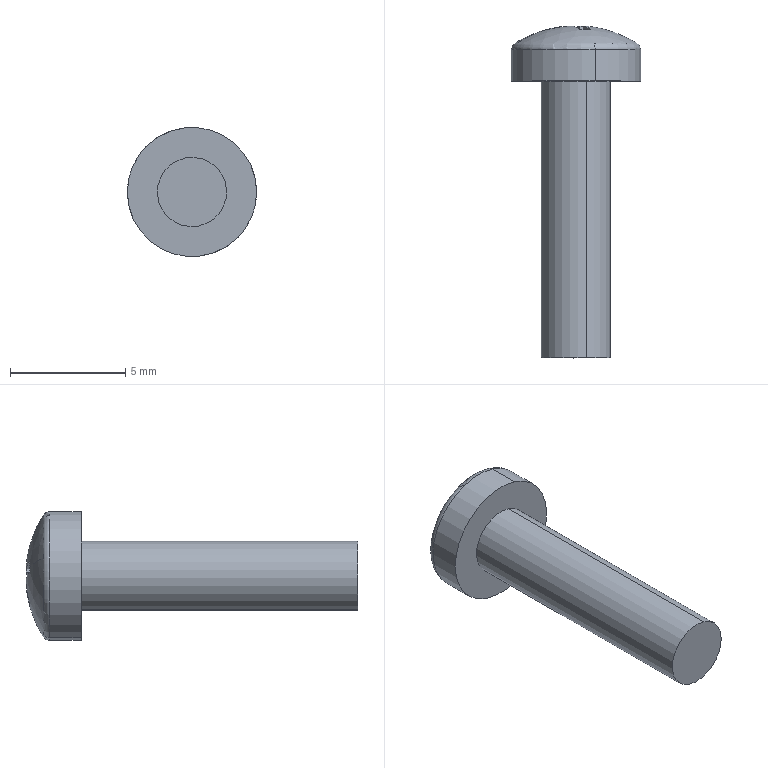Component | SolidWorks | pan cross head_am_pkg-1 | 1 solid | 23 faces | box 5.6 x 14.39 x 5.6 mm | volume 132 mm3 | plane 15 | cylinder 4 | torus 2 | sphere 2 | commonest cylinder face diameters 5.6 x2 3 x2
STEP:
#1=COLOUR_RGB('',0.7922,0.8196,0.9333);
#2=FILL_AREA_STYLE_COLOUR('',#1);
#3=FILL_AREA_STYLE('',(#2));
#4=SURFACE_STYLE_FILL_AREA(#3);
#5=SURFACE_SIDE_STYLE('',(#4));
#6=SURFACE_STYLE_USAGE(.BOTH.,#5);
#7=PRESENTATION_STYLE_ASSIGNMENT((#6));
#8=CARTESIAN_POINT('',(0.5678,0.5654,-0.7057));
#9=VERTEX_POINT('',#8);
#10=CARTESIAN_POINT('',(0.633,0.5654,-0.4951));
#11=VERTEX_POINT('',#10);
#12=CARTESIAN_POINT('',(0.6004,0.5654,-0.6004));
#13=DIRECTION('',(0.,1.,-0.));
#14=DIRECTION('',(-0.2959,0.,-0.9552));
#15=AXIS2_PLACEMENT_3D('',#12,#13,#14);
#16=CIRCLE('',#15,0.1102);
#17=EDGE_CURVE('',#9,#11,#16,.T.);
#18=ORIENTED_EDGE('',*,*,#17,.T.);
#19=CARTESIAN_POINT('',(0.6312,0.5766,-0.5011));
#20=VERTEX_POINT('',#19);
#21=CARTESIAN_POINT('',(0.6291,0.5654,-0.5077));
#22=DIRECTION('',(-0.9552,0.,0.2959));
#23=DIRECTION('',(0.2959,0.,0.9552));
#24=AXIS2_PLACEMENT_3D('',#21,#22,#23);
#25=CIRCLE('',#24,0.01323);
#26=EDGE_CURVE('',#11,#20,#25,.T.);
#27=ORIENTED_EDGE('',*,*,#26,.T.);
#28=CARTESIAN_POINT('',(0.5011,0.5766,-0.5696));
#29=VERTEX_POINT('',#28);
#30=CARTESIAN_POINT('',(0.6004,0.5766,-0.6004));
#31=DIRECTION('',(0.,1.,-0.));
#32=DIRECTION('',(-0.2959,0.,-0.9552));
#33=AXIS2_PLACEMENT_3D('',#30,#31,#32);
#34=CIRCLE('',#33,0.104);
#35=EDGE_CURVE('',#29,#20,#34,.T.);
#36=ORIENTED_EDGE('',*,*,#35,.F.);
#37=CARTESIAN_POINT('',(0.5696,0.5766,-0.6997));
#38=VERTEX_POINT('',#37);
#39=CARTESIAN_POINT('',(0.6004,0.5766,-0.6004));
#40=DIRECTION('',(0.,1.,-0.));
#41=DIRECTION('',(-0.2959,0.,-0.9552));
#42=AXIS2_PLACEMENT_3D('',#39,#40,#41);
#43=CIRCLE('',#42,0.104);
#44=EDGE_CURVE('',#38,#29,#43,.T.);
#45=ORIENTED_EDGE('',*,*,#44,.F.);
#46=CARTESIAN_POINT('',(0.5717,0.5654,-0.6931));
#47=DIRECTION('',(0.9552,-0.,-0.2959));
#48=DIRECTION('',(-0.2959,0.,-0.9552));
#49=AXIS2_PLACEMENT_3D('',#46,#47,#48);
#50=CIRCLE('',#49,0.01323);
#51=EDGE_CURVE('',#9,#38,#50,.T.);
#52=ORIENTED_EDGE('',*,*,#51,.F.);
#53=EDGE_LOOP('',(#18,#27,#36,#45,#52));
#54=FACE_OUTER_BOUND('',#53,.T.);
#55=CARTESIAN_POINT('',(0.6004,0.5654,-0.6004));
#56=DIRECTION('',(0.,1.,-0.));
#57=DIRECTION('',(-0.2959,-0.,-0.9552));
#58=AXIS2_PLACEMENT_3D('',#55,#56,#57);
#59=TOROIDAL_SURFACE('',#58,0.09701,0.01323);
#60=ADVANCED_FACE('',(#54),#59,.T.);
#61=CARTESIAN_POINT('',(0.5678,0.5118,-0.7057));
#62=VERTEX_POINT('',#61);
#63=CARTESIAN_POINT('',(0.633,0.5118,-0.4951));
#64=VERTEX_POINT('',#63);
#65=CARTESIAN_POINT('',(0.6004,0.5118,-0.6004));
#66=DIRECTION('',(0.,1.,-0.));
#67=DIRECTION('',(-0.2959,0.,-0.9552));
#68=AXIS2_PLACEMENT_3D('',#65,#66,#67);
#69=CIRCLE('',#68,0.1102);
#70=EDGE_CURVE('',#62,#64,#69,.T.);
#71=ORIENTED_EDGE('',*,*,#70,.T.);
#72=CARTESIAN_POINT('',(0.633,1.606,-0.4951));
#73=DIRECTION('',(0.,1.,-0.));
#74=VECTOR('',#73,39.37);
#75=LINE('',#72,#74);
#76=EDGE_CURVE('',#64,#11,#75,.T.);
#77=ORIENTED_EDGE('',*,*,#76,.T.);
#78=ORIENTED_EDGE('',*,*,#17,.F.);
#79=CARTESIAN_POINT('',(0.5678,1.606,-0.7057));
#80=DIRECTION('',(0.,1.,-0.));
#81=VECTOR('',#80,39.37);
#82=LINE('',#79,#81);
#83=EDGE_CURVE('',#62,#9,#82,.T.);
#84=ORIENTED_EDGE('',*,*,#83,.F.);
#85=EDGE_LOOP('',(#71,#77,#78,#84));
#86=FACE_OUTER_BOUND('',#85,.T.);
#87=CARTESIAN_POINT('',(0.6004,1.606,-0.6004));
#88=DIRECTION('',(0.,1.,-0.));
#89=DIRECTION('',(-0.2959,0.,-0.9552));
#90=AXIS2_PLACEMENT_3D('',#87,#88,#89);
#91=CYLINDRICAL_SURFACE('',#90,0.1102);
#92=ADVANCED_FACE('',(#86),#91,.T.);
#93=CARTESIAN_POINT('',(0.5829,0.03937,-0.6568));
#94=VERTEX_POINT('',#93);
#95=CARTESIAN_POINT('',(0.6179,0.03937,-0.544));
#96=VERTEX_POINT('',#95);
#97=CARTESIAN_POINT('',(0.6004,0.03937,-0.6004));
#98=DIRECTION('',(0.,1.,-0.));
#99=DIRECTION('',(-0.2959,-0.,-0.9552));
#100=AXIS2_PLACEMENT_3D('',#97,#98,#99);
#101=CIRCLE('',#100,0.05906);
#102=EDGE_CURVE('',#94,#96,#101,.T.);
#103=ORIENTED_EDGE('',*,*,#102,.T.);
#104=CARTESIAN_POINT('',(0.6179,0.5118,-0.544));
#105=VERTEX_POINT('',#104);
#106=CARTESIAN_POINT('',(0.6179,1.606,-0.544));
#107=DIRECTION('',(0.,1.,-0.));
#108=VECTOR('',#107,39.37);
#109=LINE('',#106,#108);
#110=EDGE_CURVE('',#96,#105,#109,.T.);
#111=ORIENTED_EDGE('',*,*,#110,.T.);
#112=CARTESIAN_POINT('',(0.5829,0.5118,-0.6568));
#113=VERTEX_POINT('',#112);
#114=CARTESIAN_POINT('',(0.6004,0.5118,-0.6004));
#115=DIRECTION('',(0.,1.,-0.));
#116=DIRECTION('',(-0.2959,0.,-0.9552));
#117=AXIS2_PLACEMENT_3D('',#114,#115,#116);
#118=CIRCLE('',#117,0.05906);
#119=EDGE_CURVE('',#113,#105,#118,.T.);
#120=ORIENTED_EDGE('',*,*,#119,.F.);
#121=CARTESIAN_POINT('',(0.5829,1.606,-0.6568));
#122=DIRECTION('',(0.,1.,-0.));
#123=VECTOR('',#122,39.37);
#124=LINE('',#121,#123);
#125=EDGE_CURVE('',#94,#113,#124,.T.);
#126=ORIENTED_EDGE('',*,*,#125,.F.);
#127=EDGE_LOOP('',(#103,#111,#120,#126));
#128=FACE_OUTER_BOUND('',#127,.T.);
#129=CARTESIAN_POINT('',(0.6004,1.606,-0.6004));
#130=DIRECTION('',(0.,1.,-0.));
#131=DIRECTION('',(-0.2959,0.,-0.9552));
#132=AXIS2_PLACEMENT_3D('',#129,#130,#131);
#133=CYLINDRICAL_SURFACE('',#132,0.05906);
#134=ADVANCED_FACE('',(#128),#133,.T.);
#135=ORIENTED_EDGE('',*,*,#35,.T.);
#136=CARTESIAN_POINT('',(0.6997,0.5766,-0.6312));
#137=VERTEX_POINT('',#136);
#138=CARTESIAN_POINT('',(0.6004,0.5766,-0.6004));
#139=DIRECTION('',(0.,1.,-0.));
#140=DIRECTION('',(-0.2959,0.,-0.9552));
#141=AXIS2_PLACEMENT_3D('',#138,#139,#140);
#142=CIRCLE('',#141,0.104);
#143=EDGE_CURVE('',#20,#137,#142,.T.);
#144=ORIENTED_EDGE('',*,*,#143,.T.);
#145=CARTESIAN_POINT('',(0.6496,0.5994,-0.6156));
#146=VERTEX_POINT('',#145);
#147=CARTESIAN_POINT('',(0.6004,0.4094,-0.6004));
#148=DIRECTION('',(0.2959,0.,0.9552));
#149=DIRECTION('',(0.9552,0.,-0.2959));
#150=AXIS2_PLACEMENT_3D('',#147,#148,#149);
#151=CIRCLE('',#150,0.1969);
#152=EDGE_CURVE('',#137,#146,#151,.T.);
#153=ORIENTED_EDGE('',*,*,#152,.T.);
#154=CARTESIAN_POINT('',(0.6524,0.5992,-0.6064));
#155=VERTEX_POINT('',#154);
#156=CARTESIAN_POINT('',(0.5508,0.4439,-0.585));
#157=DIRECTION('',(0.7954,-0.5538,-0.2464));
#158=DIRECTION('',(-0.529,-0.8327,0.1639));
#159=AXIS2_PLACEMENT_3D('',#156,#157,#158);
#160=CIRCLE('',#159,0.1867);
#161=EDGE_CURVE('',#146,#155,#160,.T.);
#162=ORIENTED_EDGE('',*,*,#161,.T.);
#163=CARTESIAN_POINT('',(0.613,0.6058,-0.5937));
#164=VERTEX_POINT('',#163);
#165=CARTESIAN_POINT('',(0.5995,0.4096,-0.6031));
#166=DIRECTION('',(-0.2952,0.06592,-0.9531));
#167=DIRECTION('',(-0.0195,-0.9978,-0.06296));
#168=AXIS2_PLACEMENT_3D('',#165,#166,#167);
#169=CIRCLE('',#168,0.1968);
#170=EDGE_CURVE('',#164,#155,#169,.T.);
#171=ORIENTED_EDGE('',*,*,#170,.F.);
#172=CARTESIAN_POINT('',(0.6248,0.5992,-0.5542));
#173=VERTEX_POINT('',#172);
#174=CARTESIAN_POINT('',(0.5977,0.4096,-0.5995));
#175=DIRECTION('',(-0.9531,0.06592,0.2952));
#176=DIRECTION('',(0.06296,0.9978,-0.0195));
#177=AXIS2_PLACEMENT_3D('',#174,#175,#176);
#178=CIRCLE('',#177,0.1968);
#179=EDGE_CURVE('',#173,#164,#178,.T.);
#180=ORIENTED_EDGE('',*,*,#179,.F.);
#181=CARTESIAN_POINT('',(0.6064,0.5992,-0.5484));
#182=VERTEX_POINT('',#181);
#183=CARTESIAN_POINT('',(0.585,0.4439,-0.6499));
#184=DIRECTION('',(0.2464,-0.5538,0.7954));
#185=DIRECTION('',(0.1639,0.8327,0.529));
#186=AXIS2_PLACEMENT_3D('',#183,#184,#185);
#187=CIRCLE('',#186,0.1867);
#188=EDGE_CURVE('',#173,#182,#187,.T.);
#189=ORIENTED_EDGE('',*,*,#188,.T.);
#190=CARTESIAN_POINT('',(0.5937,0.6058,-0.5878));
#191=VERTEX_POINT('',#190);
#192=CARTESIAN_POINT('',(0.6031,0.4096,-0.6012));
#193=DIRECTION('',(0.9531,0.06592,-0.2952));
#194=DIRECTION('',(0.06296,-0.9978,-0.0195));
#195=AXIS2_PLACEMENT_3D('',#192,#193,#194);
#196=CIRCLE('',#195,0.1968);
#197=EDGE_CURVE('',#191,#182,#196,.T.);
#198=ORIENTED_EDGE('',*,*,#197,.F.);
#199=CARTESIAN_POINT('',(0.5542,0.5992,-0.5759));
#200=VERTEX_POINT('',#199);
#201=CARTESIAN_POINT('',(0.5995,0.4096,-0.6031));
#202=DIRECTION('',(-0.2952,0.06592,-0.9531));
#203=DIRECTION('',(-0.0195,-0.9978,-0.06296));
#204=AXIS2_PLACEMENT_3D('',#201,#202,#203);
#205=CIRCLE('',#204,0.1968);
#206=EDGE_CURVE('',#200,#191,#205,.T.);
#207=ORIENTED_EDGE('',*,*,#206,.F.);
#208=CARTESIAN_POINT('',(0.5512,0.5994,-0.5851));
#209=VERTEX_POINT('',#208);
#210=CARTESIAN_POINT('',(0.6499,0.4439,-0.6157));
#211=DIRECTION('',(-0.7954,-0.5538,0.2464));
#212=DIRECTION('',(-0.529,0.8327,0.1639));
#213=AXIS2_PLACEMENT_3D('',#210,#211,#212);
#214=CIRCLE('',#213,0.1867);
#215=EDGE_CURVE('',#200,#209,#214,.T.);
#216=ORIENTED_EDGE('',*,*,#215,.T.);
#217=CARTESIAN_POINT('',(0.6004,0.4094,-0.6004));
#218=DIRECTION('',(-0.2959,-0.,-0.9552));
#219=DIRECTION('',(-0.9552,0.,0.2959));
#220=AXIS2_PLACEMENT_3D('',#217,#218,#219);
#221=CIRCLE('',#220,0.1969);
#222=EDGE_CURVE('',#29,#209,#221,.T.);
#223=ORIENTED_EDGE('',*,*,#222,.F.);
#224=EDGE_LOOP('',(#135,#144,#153,#162,#171,#180,#189,#198,#207,#216,#223));
#225=FACE_OUTER_BOUND('',#224,.T.);
#226=CARTESIAN_POINT('',(0.6004,0.4094,-0.6004));
#227=DIRECTION('',(0.2959,0.,0.9552));
#228=DIRECTION('',(-0.9552,0.,0.2959));
#229=AXIS2_PLACEMENT_3D('',#226,#227,#228);
#230=SPHERICAL_SURFACE('',#229,0.1969);
#231=ADVANCED_FACE('',(#225),#230,.T.);
#232=ORIENTED_EDGE('',*,*,#152,.F.);
#233=CARTESIAN_POINT('',(0.6004,0.5766,-0.6004));
#234=DIRECTION('',(0.,1.,-0.));
#235=DIRECTION('',(-0.2959,0.,-0.9552));
#236=AXIS2_PLACEMENT_3D('',#233,#234,#235);
#237=CIRCLE('',#236,0.104);
#238=EDGE_CURVE('',#137,#38,#237,.T.);
#239=ORIENTED_EDGE('',*,*,#238,.T.);
#240=ORIENTED_EDGE('',*,*,#44,.T.);
#241=ORIENTED_EDGE('',*,*,#222,.T.);
#242=CARTESIAN_POINT('',(0.5484,0.5992,-0.5944));
#243=VERTEX_POINT('',#242);
#244=CARTESIAN_POINT('',(0.6499,0.4439,-0.6157));
#245=DIRECTION('',(-0.7954,-0.5538,0.2464));
#246=DIRECTION('',(-0.529,0.8327,0.1639));
#247=AXIS2_PLACEMENT_3D('',#244,#245,#246);
#248=CIRCLE('',#247,0.1867);
#249=EDGE_CURVE('',#209,#243,#248,.T.);
#250=ORIENTED_EDGE('',*,*,#249,.T.);
#251=CARTESIAN_POINT('',(0.5878,0.6058,-0.6071));
#252=VERTEX_POINT('',#251);
#253=CARTESIAN_POINT('',(0.6012,0.4096,-0.5977));
#254=DIRECTION('',(0.2952,0.06592,0.9531));
#255=DIRECTION('',(-0.0195,0.9978,-0.06296));
#256=AXIS2_PLACEMENT_3D('',#253,#254,#255);
#257=CIRCLE('',#256,0.1968);
#258=EDGE_CURVE('',#252,#243,#257,.T.);
#259=ORIENTED_EDGE('',*,*,#258,.F.);
#260=CARTESIAN_POINT('',(0.5759,0.5992,-0.6466));
#261=VERTEX_POINT('',#260);
#262=CARTESIAN_POINT('',(0.6031,0.4096,-0.6012));
#263=DIRECTION('',(0.9531,0.06592,-0.2952));
#264=DIRECTION('',(0.06296,-0.9978,-0.0195));
#265=AXIS2_PLACEMENT_3D('',#262,#263,#264);
#266=CIRCLE('',#265,0.1968);
#267=EDGE_CURVE('',#261,#252,#266,.T.);
#268=ORIENTED_EDGE('',*,*,#267,.F.);
#269=CARTESIAN_POINT('',(0.5944,0.5992,-0.6524));
#270=VERTEX_POINT('',#269);
#271=CARTESIAN_POINT('',(0.6157,0.4439,-0.5508));
#272=DIRECTION('',(-0.2464,-0.5538,-0.7954));
#273=DIRECTION('',(0.1639,-0.8327,0.529));
#274=AXIS2_PLACEMENT_3D('',#271,#272,#273);
#275=CIRCLE('',#274,0.1867);
#276=EDGE_CURVE('',#261,#270,#275,.T.);
#277=ORIENTED_EDGE('',*,*,#276,.T.);
#278=CARTESIAN_POINT('',(0.6071,0.6058,-0.613));
#279=VERTEX_POINT('',#278);
#280=CARTESIAN_POINT('',(0.5977,0.4096,-0.5995));
#281=DIRECTION('',(-0.9531,0.06592,0.2952));
#282=DIRECTION('',(0.06296,0.9978,-0.0195));
#283=AXIS2_PLACEMENT_3D('',#280,#281,#282);
#284=CIRCLE('',#283,0.1968);
#285=EDGE_CURVE('',#279,#270,#284,.T.);
#286=ORIENTED_EDGE('',*,*,#285,.F.);
#287=CARTESIAN_POINT('',(0.6466,0.5992,-0.6248));
#288=VERTEX_POINT('',#287);
#289=CARTESIAN_POINT('',(0.6012,0.4096,-0.5977));
#290=DIRECTION('',(0.2952,0.06592,0.9531));
#291=DIRECTION('',(-0.0195,0.9978,-0.06296));
#292=AXIS2_PLACEMENT_3D('',#289,#290,#291);
#293=CIRCLE('',#292,0.1968);
#294=EDGE_CURVE('',#288,#279,#293,.T.);
#295=ORIENTED_EDGE('',*,*,#294,.F.);
#296=CARTESIAN_POINT('',(0.5508,0.4439,-0.585));
#297=DIRECTION('',(0.7954,-0.5538,-0.2464));
#298=DIRECTION('',(-0.529,-0.8327,0.1639));
#299=AXIS2_PLACEMENT_3D('',#296,#297,#298);
#300=CIRCLE('',#299,0.1867);
#301=EDGE_CURVE('',#288,#146,#300,.T.);
#302=ORIENTED_EDGE('',*,*,#301,.T.);
#303=EDGE_LOOP('',(#232,#239,#240,#241,#250,#259,#268,#277,#286,#295,#302));
#304=FACE_OUTER_BOUND('',#303,.T.);
#305=CARTESIAN_POINT('',(0.6004,0.4094,-0.6004));
#306=DIRECTION('',(0.2959,0.,0.9552));
#307=DIRECTION('',(-0.9552,0.,0.2959));
#308=AXIS2_PLACEMENT_3D('',#305,#306,#307);
#309=SPHERICAL_SURFACE('',#308,0.1969);
#310=ADVANCED_FACE('',(#304),#309,.T.);
#311=ORIENTED_EDGE('',*,*,#206,.T.);
#312=CARTESIAN_POINT('',(0.5971,0.5296,-0.5941));
#313=VERTEX_POINT('',#312);
#314=CARTESIAN_POINT('',(0.5974,0.5216,-0.5947));
#315=DIRECTION('',(0.04337,-0.9957,-0.08229));
#316=VECTOR('',#315,39.37);
#317=LINE('',#314,#316);
#318=EDGE_CURVE('',#191,#313,#317,.T.);
#319=ORIENTED_EDGE('',*,*,#318,.T.);
#320=CARTESIAN_POINT('',(0.5498,0.6063,-0.5741));
#321=DIRECTION('',(0.5119,-0.8314,-0.2161));
#322=VECTOR('',#321,39.37);
#323=LINE('',#320,#322);
#324=EDGE_CURVE('',#200,#313,#323,.T.);
#325=ORIENTED_EDGE('',*,*,#324,.F.);
#326=EDGE_LOOP('',(#311,#319,#325));
#327=FACE_OUTER_BOUND('',#326,.T.);
#328=CARTESIAN_POINT('',(0.6017,0.5219,-0.596));
#329=DIRECTION('',(-0.2952,0.06592,-0.9531));
#330=DIRECTION('',(-0.0195,-0.9978,-0.06296));
#331=AXIS2_PLACEMENT_3D('',#328,#329,#330);
#332=PLANE('',#331);
#333=ADVANCED_FACE('',(#327),#332,.T.);
#334=CARTESIAN_POINT('',(0.6067,0.5296,-0.5971));
#335=VERTEX_POINT('',#334);
#336=CARTESIAN_POINT('',(0.657,0.6063,-0.6073));
#337=DIRECTION('',(-0.5444,-0.8314,0.1111));
#338=VECTOR('',#337,39.37);
#339=LINE('',#336,#338);
#340=EDGE_CURVE('',#155,#335,#339,.T.);
#341=ORIENTED_EDGE('',*,*,#340,.T.);
#342=CARTESIAN_POINT('',(0.6061,0.5216,-0.5974));
#343=DIRECTION('',(0.08229,0.9957,0.04337));
#344=VECTOR('',#343,39.37);
#345=LINE('',#342,#344);
#346=EDGE_CURVE('',#335,#164,#345,.T.);
#347=ORIENTED_EDGE('',*,*,#346,.T.);
#348=ORIENTED_EDGE('',*,*,#170,.T.);
#349=EDGE_LOOP('',(#341,#347,#348));
#350=FACE_OUTER_BOUND('',#349,.T.);
#351=CARTESIAN_POINT('',(0.6017,0.5219,-0.596));
#352=DIRECTION('',(-0.2952,0.06592,-0.9531));
#353=DIRECTION('',(-0.0195,-0.9978,-0.06296));
#354=AXIS2_PLACEMENT_3D('',#351,#352,#353);
#355=PLANE('',#354);
#356=ADVANCED_FACE('',(#350),#355,.T.);
#357=CARTESIAN_POINT('',(0.5941,0.5296,-0.6037));
#358=VERTEX_POINT('',#357);
#359=CARTESIAN_POINT('',(0.5438,0.6063,-0.5935));
#360=DIRECTION('',(0.5444,-0.8314,-0.1111));
#361=VECTOR('',#360,39.37);
#362=LINE('',#359,#361);
#363=EDGE_CURVE('',#243,#358,#362,.T.);
#364=ORIENTED_EDGE('',*,*,#363,.T.);
#365=CARTESIAN_POINT('',(0.5947,0.5216,-0.6034));
#366=DIRECTION('',(-0.08229,0.9957,-0.04337));
#367=VECTOR('',#366,39.37);
#368=LINE('',#365,#367);
#369=EDGE_CURVE('',#358,#252,#368,.T.);
#370=ORIENTED_EDGE('',*,*,#369,.T.);
#371=ORIENTED_EDGE('',*,*,#258,.T.);
#372=EDGE_LOOP('',(#364,#370,#371));
#373=FACE_OUTER_BOUND('',#372,.T.);
#374=CARTESIAN_POINT('',(0.599,0.5219,-0.6048));
#375=DIRECTION('',(0.2952,0.06592,0.9531));
#376=DIRECTION('',(-0.0195,0.9978,-0.06296));
#377=AXIS2_PLACEMENT_3D('',#374,#375,#376);
#378=PLANE('',#377);
#379=ADVANCED_FACE('',(#373),#378,.T.);
#380=ORIENTED_EDGE('',*,*,#294,.T.);
#381=CARTESIAN_POINT('',(0.6037,0.5296,-0.6067));
#382=VERTEX_POINT('',#381);
#383=CARTESIAN_POINT('',(0.6034,0.5216,-0.6061));
#384=DIRECTION('',(-0.04337,-0.9957,0.08229));
#385=VECTOR('',#384,39.37);
#386=LINE('',#383,#385);
#387=EDGE_CURVE('',#279,#382,#386,.T.);
#388=ORIENTED_EDGE('',*,*,#387,.T.);
#389=CARTESIAN_POINT('',(0.651,0.6063,-0.6267));
#390=DIRECTION('',(-0.5119,-0.8314,0.2161));
#391=VECTOR('',#390,39.37);
#392=LINE('',#389,#391);
#393=EDGE_CURVE('',#288,#382,#392,.T.);
#394=ORIENTED_EDGE('',*,*,#393,.F.);
#395=EDGE_LOOP('',(#380,#388,#394));
#396=FACE_OUTER_BOUND('',#395,.T.);
#397=CARTESIAN_POINT('',(0.599,0.5219,-0.6048));
#398=DIRECTION('',(0.2952,0.06592,0.9531));
#399=DIRECTION('',(-0.0195,0.9978,-0.06296));
#400=AXIS2_PLACEMENT_3D('',#397,#398,#399);
#401=PLANE('',#400);
#402=ADVANCED_FACE('',(#396),#401,.T.);
#403=ORIENTED_EDGE('',*,*,#110,.F.);
#404=CARTESIAN_POINT('',(0.6004,0.03937,-0.6004));
#405=DIRECTION('',(0.,1.,-0.));
#406=DIRECTION('',(-0.2959,-0.,-0.9552));
#407=AXIS2_PLACEMENT_3D('',#404,#405,#406);
#408=CIRCLE('',#407,0.05906);
#409=EDGE_CURVE('',#96,#94,#408,.T.);
#410=ORIENTED_EDGE('',*,*,#409,.T.);
#411=ORIENTED_EDGE('',*,*,#125,.T.);
#412=CARTESIAN_POINT('',(0.6004,0.5118,-0.6004));
#413=DIRECTION('',(0.,1.,-0.));
#414=DIRECTION('',(-0.2959,0.,-0.9552));
#415=AXIS2_PLACEMENT_3D('',#412,#413,#414);
#416=CIRCLE('',#415,0.05906);
#417=EDGE_CURVE('',#105,#113,#416,.T.);
#418=ORIENTED_EDGE('',*,*,#417,.F.);
#419=EDGE_LOOP('',(#403,#410,#411,#418));
#420=FACE_OUTER_BOUND('',#419,.T.);
#421=CARTESIAN_POINT('',(0.6004,1.606,-0.6004));
#422=DIRECTION('',(0.,1.,-0.));
#423=DIRECTION('',(-0.2959,0.,-0.9552));
#424=AXIS2_PLACEMENT_3D('',#421,#422,#423);
#425=CYLINDRICAL_SURFACE('',#424,0.05906);
#426=ADVANCED_FACE('',(#420),#425,.T.);
#427=ORIENTED_EDGE('',*,*,#70,.F.);
#428=CARTESIAN_POINT('',(0.6004,0.5118,-0.6004));
#429=DIRECTION('',(0.,1.,-0.));
#430=DIRECTION('',(-0.2959,0.,-0.9552));
#431=AXIS2_PLACEMENT_3D('',#428,#429,#430);
#432=CIRCLE('',#431,0.1102);
#433=EDGE_CURVE('',#64,#62,#432,.T.);
#434=ORIENTED_EDGE('',*,*,#433,.F.);
#435=EDGE_LOOP('',(#427,#434));
#436=FACE_OUTER_BOUND('',#435,.T.);
#437=ORIENTED_EDGE('',*,*,#119,.T.);
#438=ORIENTED_EDGE('',*,*,#417,.T.);
#439=EDGE_LOOP('',(#437,#438));
#440=FACE_BOUND('',#439,.T.);
#441=CARTESIAN_POINT('',(0.544,0.5118,-0.5829));
#442=DIRECTION('',(0.,1.,-0.));
#443=DIRECTION('',(-0.2959,-0.,-0.9552));
#444=AXIS2_PLACEMENT_3D('',#441,#442,#443);
#445=PLANE('',#444);
#446=ADVANCED_FACE('',(#436,#440),#445,.F.);
#447=ORIENTED_EDGE('',*,*,#76,.F.);
#448=ORIENTED_EDGE('',*,*,#433,.T.);
#449=ORIENTED_EDGE('',*,*,#83,.T.);
#450=CARTESIAN_POINT('',(0.6004,0.5654,-0.6004));
#451=DIRECTION('',(0.,1.,-0.));
#452=DIRECTION('',(-0.2959,0.,-0.9552));
#453=AXIS2_PLACEMENT_3D('',#450,#451,#452);
#454=CIRCLE('',#453,0.1102);
#455=EDGE_CURVE('',#11,#9,#454,.T.);
#456=ORIENTED_EDGE('',*,*,#455,.F.);
#457=EDGE_LOOP('',(#447,#448,#449,#456));
#458=FACE_OUTER_BOUND('',#457,.T.);
#459=CARTESIAN_POINT('',(0.6004,1.606,-0.6004));
#460=DIRECTION('',(0.,1.,-0.));
#461=DIRECTION('',(-0.2959,0.,-0.9552));
#462=AXIS2_PLACEMENT_3D('',#459,#460,#461);
#463=CYLINDRICAL_SURFACE('',#462,0.1102);
#464=ADVANCED_FACE('',(#458),#463,.T.);
#465=ORIENTED_EDGE('',*,*,#26,.F.);
#466=ORIENTED_EDGE('',*,*,#455,.T.);
#467=ORIENTED_EDGE('',*,*,#51,.T.);
#468=ORIENTED_EDGE('',*,*,#238,.F.);
#469=ORIENTED_EDGE('',*,*,#143,.F.);
#470=EDGE_LOOP('',(#465,#466,#467,#468,#469));
#471=FACE_OUTER_BOUND('',#470,.T.);
#472=CARTESIAN_POINT('',(0.6004,0.5654,-0.6004));
#473=DIRECTION('',(0.,1.,-0.));
#474=DIRECTION('',(-0.2959,-0.,-0.9552));
#475=AXIS2_PLACEMENT_3D('',#472,#473,#474);
#476=TOROIDAL_SURFACE('',#475,0.09701,0.01323);
#477=ADVANCED_FACE('',(#471),#476,.T.);
#478=ORIENTED_EDGE('',*,*,#102,.F.);
#479=ORIENTED_EDGE('',*,*,#409,.F.);
#480=EDGE_LOOP('',(#478,#479));
#481=FACE_OUTER_BOUND('',#480,.T.);
#482=CARTESIAN_POINT('',(0.544,0.03937,-0.5829));
#483=DIRECTION('',(-0.,-1.,0.));
#484=DIRECTION('',(0.2959,0.,0.9552));
#485=AXIS2_PLACEMENT_3D('',#482,#483,#484);
#486=PLANE('',#485);
#487=ADVANCED_FACE('',(#481),#486,.T.);
#488=ORIENTED_EDGE('',*,*,#324,.T.);
#489=CARTESIAN_POINT('',(0.5941,0.5296,-0.6037));
#490=DIRECTION('',(0.2959,0.,0.9552));
#491=VECTOR('',#490,39.37);
#492=LINE('',#489,#491);
#493=EDGE_CURVE('',#358,#313,#492,.T.);
#494=ORIENTED_EDGE('',*,*,#493,.F.);
#495=ORIENTED_EDGE('',*,*,#363,.F.);
#496=ORIENTED_EDGE('',*,*,#249,.F.);
#497=ORIENTED_EDGE('',*,*,#215,.F.);
#498=EDGE_LOOP('',(#488,#494,#495,#496,#497));
#499=FACE_OUTER_BOUND('',#498,.T.);
#500=CARTESIAN_POINT('',(0.5941,0.5296,-0.6037));
#501=DIRECTION('',(-0.7954,-0.5538,0.2464));
#502=DIRECTION('',(-0.529,0.8327,0.1639));
#503=AXIS2_PLACEMENT_3D('',#500,#501,#502);
#504=PLANE('',#503);
#505=ADVANCED_FACE('',(#499),#504,.F.);
#506=ORIENTED_EDGE('',*,*,#393,.T.);
#507=CARTESIAN_POINT('',(0.6067,0.5296,-0.5971));
#508=DIRECTION('',(-0.2959,-0.,-0.9552));
#509=VECTOR('',#508,39.37);
#510=LINE('',#507,#509);
#511=EDGE_CURVE('',#335,#382,#510,.T.);
#512=ORIENTED_EDGE('',*,*,#511,.F.);
#513=ORIENTED_EDGE('',*,*,#340,.F.);
#514=ORIENTED_EDGE('',*,*,#161,.F.);
#515=ORIENTED_EDGE('',*,*,#301,.F.);
#516=EDGE_LOOP('',(#506,#512,#513,#514,#515));
#517=FACE_OUTER_BOUND('',#516,.T.);
#518=CARTESIAN_POINT('',(0.6067,0.5296,-0.5971));
#519=DIRECTION('',(0.7954,-0.5538,-0.2464));
#520=DIRECTION('',(-0.529,-0.8327,0.1639));
#521=AXIS2_PLACEMENT_3D('',#518,#519,#520);
#522=PLANE('',#521);
#523=ADVANCED_FACE('',(#517),#522,.F.);
#524=CARTESIAN_POINT('',(0.6067,0.5296,-0.5971));
#525=DIRECTION('',(-0.9552,0.,0.2959));
#526=VECTOR('',#525,39.37);
#527=LINE('',#524,#526);
#528=EDGE_CURVE('',#335,#313,#527,.T.);
#529=ORIENTED_EDGE('',*,*,#528,.F.);
#530=ORIENTED_EDGE('',*,*,#511,.T.);
#531=CARTESIAN_POINT('',(0.5941,0.5296,-0.6037));
#532=DIRECTION('',(0.9552,-0.,-0.2959));
#533=VECTOR('',#532,39.37);
#534=LINE('',#531,#533);
#535=EDGE_CURVE('',#358,#382,#534,.T.);
#536=ORIENTED_EDGE('',*,*,#535,.F.);
#537=ORIENTED_EDGE('',*,*,#493,.T.);
#538=EDGE_LOOP('',(#529,#530,#536,#537));
#539=FACE_OUTER_BOUND('',#538,.T.);
#540=CARTESIAN_POINT('',(0.5971,0.5296,-0.5941));
#541=DIRECTION('',(0.,1.,-0.));
#542=DIRECTION('',(-0.2959,-0.,-0.9552));
#543=AXIS2_PLACEMENT_3D('',#540,#541,#542);
#544=PLANE('',#543);
#545=ADVANCED_FACE('',(#539),#544,.T.);
#546=CARTESIAN_POINT('',(0.6267,0.6063,-0.5498));
#547=DIRECTION('',(-0.2161,-0.8314,-0.5119));
#548=VECTOR('',#547,39.37);
#549=LINE('',#546,#548);
#550=EDGE_CURVE('',#173,#335,#549,.T.);
#551=ORIENTED_EDGE('',*,*,#550,.T.);
#552=ORIENTED_EDGE('',*,*,#528,.T.);
#553=CARTESIAN_POINT('',(0.6073,0.6063,-0.5438));
#554=DIRECTION('',(-0.1111,-0.8314,-0.5444));
#555=VECTOR('',#554,39.37);
#556=LINE('',#553,#555);
#557=EDGE_CURVE('',#182,#313,#556,.T.);
#558=ORIENTED_EDGE('',*,*,#557,.F.);
#559=ORIENTED_EDGE('',*,*,#188,.F.);
#560=EDGE_LOOP('',(#551,#552,#558,#559));
#561=FACE_OUTER_BOUND('',#560,.T.);
#562=CARTESIAN_POINT('',(0.5971,0.5296,-0.5941));
#563=DIRECTION('',(0.2464,-0.5538,0.7954));
#564=DIRECTION('',(-0.1639,-0.8327,-0.529));
#565=AXIS2_PLACEMENT_3D('',#562,#563,#564);
#566=PLANE('',#565);
#567=ADVANCED_FACE('',(#561),#566,.F.);
#568=ORIENTED_EDGE('',*,*,#179,.T.);
#569=ORIENTED_EDGE('',*,*,#346,.F.);
#570=ORIENTED_EDGE('',*,*,#550,.F.);
#571=EDGE_LOOP('',(#568,#569,#570));
#572=FACE_OUTER_BOUND('',#571,.T.);
#573=CARTESIAN_POINT('',(0.6048,0.5219,-0.6017));
#574=DIRECTION('',(-0.9531,0.06592,0.2952));
#575=DIRECTION('',(0.06296,0.9978,-0.0195));
#576=AXIS2_PLACEMENT_3D('',#573,#574,#575);
#577=PLANE('',#576);
#578=ADVANCED_FACE('',(#572),#577,.T.);
#579=ORIENTED_EDGE('',*,*,#197,.T.);
#580=ORIENTED_EDGE('',*,*,#557,.T.);
#581=ORIENTED_EDGE('',*,*,#318,.F.);
#582=EDGE_LOOP('',(#579,#580,#581));
#583=FACE_OUTER_BOUND('',#582,.T.);
#584=CARTESIAN_POINT('',(0.596,0.5219,-0.599));
#585=DIRECTION('',(0.9531,0.06592,-0.2952));
#586=DIRECTION('',(0.06296,-0.9978,-0.0195));
#587=AXIS2_PLACEMENT_3D('',#584,#585,#586);
#588=PLANE('',#587);
#589=ADVANCED_FACE('',(#583),#588,.T.);
#590=CARTESIAN_POINT('',(0.5741,0.6063,-0.651));
#591=DIRECTION('',(0.2161,-0.8314,0.5119));
#592=VECTOR('',#591,39.37);
#593=LINE('',#590,#592);
#594=EDGE_CURVE('',#261,#358,#593,.T.);
#595=ORIENTED_EDGE('',*,*,#594,.T.);
#596=ORIENTED_EDGE('',*,*,#535,.T.);
#597=CARTESIAN_POINT('',(0.5935,0.6063,-0.657));
#598=DIRECTION('',(0.1111,-0.8314,0.5444));
#599=VECTOR('',#598,39.37);
#600=LINE('',#597,#599);
#601=EDGE_CURVE('',#270,#382,#600,.T.);
#602=ORIENTED_EDGE('',*,*,#601,.F.);
#603=ORIENTED_EDGE('',*,*,#276,.F.);
#604=EDGE_LOOP('',(#595,#596,#602,#603));
#605=FACE_OUTER_BOUND('',#604,.T.);
#606=CARTESIAN_POINT('',(0.6037,0.5296,-0.6067));
#607=DIRECTION('',(-0.2464,-0.5538,-0.7954));
#608=DIRECTION('',(-0.1639,0.8327,-0.529));
#609=AXIS2_PLACEMENT_3D('',#606,#607,#608);
#610=PLANE('',#609);
#611=ADVANCED_FACE('',(#605),#610,.F.);
#612=ORIENTED_EDGE('',*,*,#267,.T.);
#613=ORIENTED_EDGE('',*,*,#369,.F.);
#614=ORIENTED_EDGE('',*,*,#594,.F.);
#615=EDGE_LOOP('',(#612,#613,#614));
#616=FACE_OUTER_BOUND('',#615,.T.);
#617=CARTESIAN_POINT('',(0.596,0.5219,-0.599));
#618=DIRECTION('',(0.9531,0.06592,-0.2952));
#619=DIRECTION('',(0.06296,-0.9978,-0.0195));
#620=AXIS2_PLACEMENT_3D('',#617,#618,#619);
#621=PLANE('',#620);
#622=ADVANCED_FACE('',(#616),#621,.T.);
#623=ORIENTED_EDGE('',*,*,#285,.T.);
#624=ORIENTED_EDGE('',*,*,#601,.T.);
#625=ORIENTED_EDGE('',*,*,#387,.F.);
#626=EDGE_LOOP('',(#623,#624,#625));
#627=FACE_OUTER_BOUND('',#626,.T.);
#628=CARTESIAN_POINT('',(0.6048,0.5219,-0.6017));
#629=DIRECTION('',(-0.9531,0.06592,0.2952));
#630=DIRECTION('',(0.06296,0.9978,-0.0195));
#631=AXIS2_PLACEMENT_3D('',#628,#629,#630);
#632=PLANE('',#631);
#633=ADVANCED_FACE('',(#627),#632,.T.);
#634=CLOSED_SHELL('',(#60,#92,#134,#231,#310,#333,#356,#379,#402,#426,#446,#464,#477,#487,#505,#523,#545,#567,#578,#589,#611,#622,#633));
#635=MANIFOLD_SOLID_BREP('',#634);
#636=STYLED_ITEM('',(#7),#635);
#637=PRESENTATION_LAYER_ASSIGNMENT('','',(#636));
#638=CARTESIAN_POINT('',(0.,0.,0.));
#639=DIRECTION('',(0.,0.,1.));
#640=DIRECTION('',(1.,0.,0.));
#641=AXIS2_PLACEMENT_3D('',#638,#639,#640);
#642=(LENGTH_UNIT()NAMED_UNIT(*)SI_UNIT($,.METRE.));
#643=LENGTH_MEASURE_WITH_UNIT(LENGTH_MEASURE(0.0254),#642);
#644=DIMENSIONAL_EXPONENTS(1.,0.,0.,0.,0.,0.,0.);
#645=(CONVERSION_BASED_UNIT('',#643)LENGTH_UNIT()NAMED_UNIT(#644));
#646=UNCERTAINTY_MEASURE_WITH_UNIT(LENGTH_MEASURE(0.00001),#645,'','');
#647=(NAMED_UNIT(*)PLANE_ANGLE_UNIT()SI_UNIT($,.RADIAN.));
#648=(NAMED_UNIT(*)SI_UNIT($,.STERADIAN.)SOLID_ANGLE_UNIT());
#649=(GEOMETRIC_REPRESENTATION_CONTEXT(3)GLOBAL_UNCERTAINTY_ASSIGNED_CONTEXT((#646))GLOBAL_UNIT_ASSIGNED_CONTEXT((#645,#647,#648))REPRESENTATION_CONTEXT('',''));
#650=ADVANCED_BREP_SHAPE_REPRESENTATION('',(#635,#641),#649);
#651=(LENGTH_UNIT()NAMED_UNIT(*)SI_UNIT($,.METRE.));
#652=LENGTH_MEASURE_WITH_UNIT(LENGTH_MEASURE(0.0254),#651);
#653=DIMENSIONAL_EXPONENTS(1.,0.,0.,0.,0.,0.,0.);
#654=(CONVERSION_BASED_UNIT('',#652)LENGTH_UNIT()NAMED_UNIT(#653));
#655=UNCERTAINTY_MEASURE_WITH_UNIT(LENGTH_MEASURE(0.00001),#654,'','');
#656=(NAMED_UNIT(*)PLANE_ANGLE_UNIT()SI_UNIT($,.RADIAN.));
#657=(NAMED_UNIT(*)SI_UNIT($,.STERADIAN.)SOLID_ANGLE_UNIT());
#658=(GEOMETRIC_REPRESENTATION_CONTEXT(3)GLOBAL_UNCERTAINTY_ASSIGNED_CONTEXT((#655))GLOBAL_UNIT_ASSIGNED_CONTEXT((#654,#656,#657))REPRESENTATION_CONTEXT('',''));
#659=MECHANICAL_DESIGN_GEOMETRIC_PRESENTATION_REPRESENTATION('',(#636),#658);